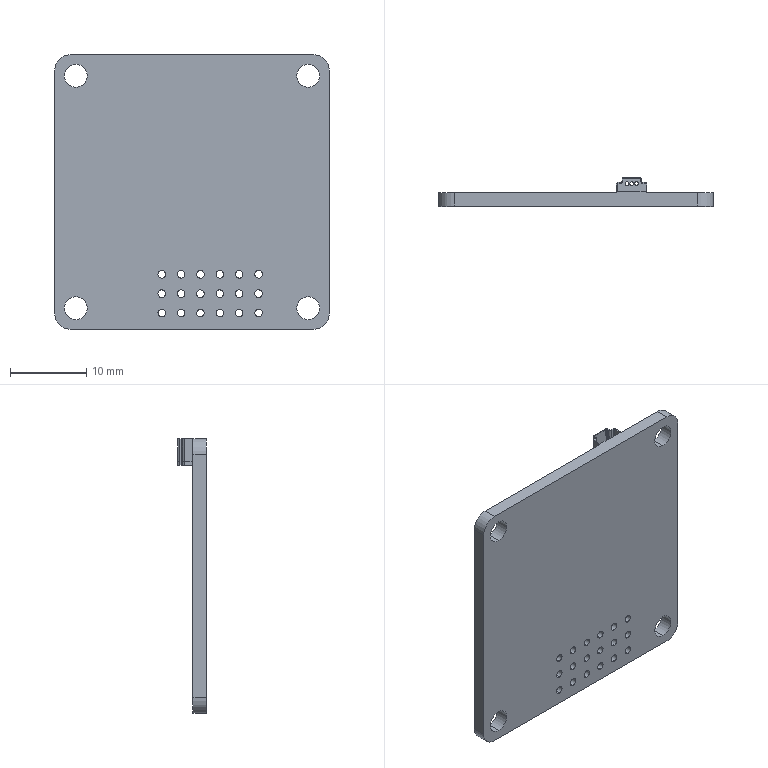Component | SolidWorks | 11.Distribution board-2 | 1 solid | 89 faces | box 36 x 3.75 x 36 mm | volume 2194 mm3 | cylinder 66 | plane 23 | commonest cylinder face diameters 1 x36 3 x8 0.486 x6 0.4 x6 4 x4 0.2 x4 0.6 x2
build123d program:
from build123d import *

# Parameters (mm, degrees)
SKETCH1_R               = 1.5
BOSS_EXTRUDE1_DEPTH     = 1.75
BOSS_EXTRUDE2_DEPTH     = 3
BOSS_EXTRUDE3_DEPTH     = 0.5
CUT_EXTRUDE1_REACH      = 39.34
SKETCH4_R               = 0.2432
CUT_EXTRUDE2_DEPTH      = 26.731
CUT_EXTRUDE2_DEPTH_BACK = 26.731
SKETCH5_R               = 0.5


with BuildPart() as part:
    # Sketch1 → Boss-Extrude1 (new body)
    with BuildSketch(Plane(origin=(0, 0, 0), x_dir=(1, 0, 0), z_dir=(0, 1, 0))):
        with BuildLine():
            Line((-16, -18), (16, -18))
            ThreePointArc((16, -18), (17.414, -17.414), (18, -16))
            Line((18, -16), (18, 16))
            ThreePointArc((18, 16), (17.414, 17.414), (16, 18))
            Line((16, 18), (-16, 18))
            ThreePointArc((-16, 18), (-17.414, 17.414), (-18, 16))
            Line((-18, 16), (-18, -16))
            ThreePointArc((-18, -16), (-17.414, -17.414), (-16, -18))
        make_face()
        with Locations(Location((-15.25, 15.25, 0), (0, 0, 270))):
            Circle(SKETCH1_R, mode=Mode.SUBTRACT)
        with Locations(Location((15.25, 15.25, 0), (0, 0, 270))):
            Circle(SKETCH1_R, mode=Mode.SUBTRACT)
        with Locations(Location((15.25, -15.25, 0), (0, 0, 270))):
            Circle(SKETCH1_R, mode=Mode.SUBTRACT)
        with Locations(Location((-15.25, -15.25, 0), (0, 0, 270))):
            Circle(SKETCH1_R, mode=Mode.SUBTRACT)
    extrude(amount=BOSS_EXTRUDE1_DEPTH)

    # Sketch2 → Boss-Extrude2 (add)
    with BuildSketch(Plane.XY.offset(18)):
        with BuildLine():
            Line((5.307, 1.75), (9.307, 1.75))
            Line((9.307, 1.75), (9.307, 2.894))
            ThreePointArc((9.307, 2.894), (9.248, 3.035), (9.107, 3.094))
            Line((9.107, 3.094), (8.767, 3.094))
            ThreePointArc((8.767, 3.094), (8.626, 3.152), (8.567, 3.294))
            Line((8.567, 3.294), (8.567, 3.55))
            ThreePointArc((8.567, 3.55), (8.508, 3.691), (8.367, 3.75))
            Line((8.367, 3.75), (6.247, 3.75))
            ThreePointArc((6.247, 3.75), (6.105, 3.691), (6.047, 3.55))
            Line((6.047, 3.55), (6.047, 3.294))
            ThreePointArc((6.047, 3.294), (5.988, 3.152), (5.847, 3.094))
            Line((5.847, 3.094), (5.507, 3.094))
            ThreePointArc((5.507, 3.094), (5.365, 3.035), (5.307, 2.894))
            Line((5.307, 2.894), (5.307, 1.75))
        make_face()
        with BuildLine():
            Line((6.247, 3.65), (8.367, 3.65))
            ThreePointArc((8.367, 3.65), (8.438, 3.621), (8.467, 3.55))
            Line((8.467, 3.55), (8.467, 3.294))
            ThreePointArc((8.467, 3.294), (8.555, 3.082), (8.767, 2.994))
            Line((8.767, 2.994), (9.107, 2.994))
            ThreePointArc((9.107, 2.994), (9.178, 2.965), (9.207, 2.894))
            Line((9.207, 2.894), (9.207, 1.85))
            Line((9.207, 1.85), (5.407, 1.85))
            Line((5.407, 1.85), (5.407, 2.894))
            ThreePointArc((5.407, 2.894), (5.436, 2.965), (5.507, 2.994))
            Line((5.507, 2.994), (5.847, 2.994))
            ThreePointArc((5.847, 2.994), (6.059, 3.082), (6.147, 3.294))
            Line((6.147, 3.294), (6.147, 3.55))
            ThreePointArc((6.147, 3.55), (6.176, 3.621), (6.247, 3.65))
        make_face(mode=Mode.SUBTRACT)
    extrude(amount=-BOSS_EXTRUDE2_DEPTH)

    # Sketch3 → Boss-Extrude3 (add)
    with BuildSketch(Plane(origin=(0, 0, 15), x_dir=(-1, 0, 0), z_dir=(0, 0, -1))):
        with BuildLine():
            Line((-5.307, 1.75), (-5.307, 2.894))
            ThreePointArc((-5.307, 2.894), (-5.365, 3.035), (-5.507, 3.094))
            Line((-5.507, 3.094), (-5.847, 3.094))
            ThreePointArc((-5.847, 3.094), (-5.988, 3.152), (-6.047, 3.294))
            Line((-6.047, 3.294), (-6.047, 3.55))
            ThreePointArc((-6.047, 3.55), (-6.105, 3.691), (-6.247, 3.75))
            Line((-6.247, 3.75), (-8.367, 3.75))
            ThreePointArc((-8.367, 3.75), (-8.508, 3.691), (-8.567, 3.55))
            Line((-8.567, 3.55), (-8.567, 3.294))
            ThreePointArc((-8.567, 3.294), (-8.626, 3.152), (-8.767, 3.094))
            Line((-8.767, 3.094), (-9.107, 3.094))
            ThreePointArc((-9.107, 3.094), (-9.248, 3.035), (-9.307, 2.894))
            Line((-9.307, 2.894), (-9.307, 1.75))
            Line((-9.307, 1.75), (-5.307, 1.75))
        make_face()
    extrude(amount=BOSS_EXTRUDE3_DEPTH)

    # Sketch4 → Cut-Extrude1 (cut, up to next)
    with BuildSketch(Plane(origin=(0, 0, 14.5), x_dir=(-1, 0, 0), z_dir=(0, 0, -1)), mode=Mode.PRIVATE) as cut_extrude1_sk1:
        with Locations((-7.307, 2.952)):
            Circle(SKETCH4_R)
    cut_extrude1_tool1 = extrude(cut_extrude1_sk1.sketch, amount=-CUT_EXTRUDE1_REACH, mode=Mode.PRIVATE) & part.part
    # Sketch4 → Cut-Extrude1 (cut, up to next)
    with BuildSketch(Plane(origin=(0, 0, 14.5), x_dir=(-1, 0, 0), z_dir=(0, 0, -1)), mode=Mode.PRIVATE) as cut_extrude1_sk2:
        with Locations((-6.69, 2.952)):
            Circle(SKETCH4_R)
    cut_extrude1_tool2 = extrude(cut_extrude1_sk2.sketch, amount=-CUT_EXTRUDE1_REACH, mode=Mode.PRIVATE) & part.part
    # Sketch4 → Cut-Extrude1 (cut, up to next)
    with BuildSketch(Plane(origin=(0, 0, 14.5), x_dir=(-1, 0, 0), z_dir=(0, 0, -1)), mode=Mode.PRIVATE) as cut_extrude1_sk3:
        with Locations((-7.932, 2.952)):
            Circle(SKETCH4_R)
    cut_extrude1_tool3 = extrude(cut_extrude1_sk3.sketch, amount=-CUT_EXTRUDE1_REACH, mode=Mode.PRIVATE) & part.part
    add(cut_extrude1_tool1.solids().sort_by_distance((7.307, 2.952, 14.5))[0], mode=Mode.SUBTRACT)
    add(cut_extrude1_tool2.solids().sort_by_distance((6.69, 2.952, 14.5))[0], mode=Mode.SUBTRACT)
    add(cut_extrude1_tool3.solids().sort_by_distance((7.932, 2.952, 14.5))[0], mode=Mode.SUBTRACT)

    # Sketch5 → Cut-Extrude2 (cut, two sides: drawn at the far end of the back side and taken through both)
    with BuildSketch(Plane.XZ.offset(-CUT_EXTRUDE2_DEPTH_BACK)):
        with Locations(Location((-3.97, -10.8, 0), (0, 0, 270))):
            Circle(SKETCH5_R)
        with Locations(Location((-3.97, -13.34, 0), (0, 0, 270))):
            Circle(SKETCH5_R)
        with Locations(Location((-3.97, -15.88, 0), (0, 0, 270))):
            Circle(SKETCH5_R)
        with Locations(Location((-1.43, -10.8, 0), (0, 0, 270))):
            Circle(SKETCH5_R)
        with Locations(Location((-1.43, -13.34, 0), (0, 0, 270))):
            Circle(SKETCH5_R)
        with Locations(Location((-1.43, -15.88, 0), (0, 0, 270))):
            Circle(SKETCH5_R)
        with Locations(Location((1.11, -10.8, 0), (0, 0, 270))):
            Circle(SKETCH5_R)
        with Locations(Location((1.11, -13.34, 0), (0, 0, 270))):
            Circle(SKETCH5_R)
        with Locations(Location((1.11, -15.88, 0), (0, 0, 270))):
            Circle(SKETCH5_R)
        with Locations(Location((3.65, -10.8, 0), (0, 0, 270))):
            Circle(SKETCH5_R)
        with Locations(Location((3.65, -13.34, 0), (0, 0, 270))):
            Circle(SKETCH5_R)
        with Locations(Location((3.65, -15.88, 0), (0, 0, 270))):
            Circle(SKETCH5_R)
        with Locations(Location((6.19, -10.8, 0), (0, 0, 270))):
            Circle(SKETCH5_R)
        with Locations(Location((6.19, -13.34, 0), (0, 0, 270))):
            Circle(SKETCH5_R)
        with Locations(Location((6.19, -15.88, 0), (0, 0, 270))):
            Circle(SKETCH5_R)
        with Locations(Location((8.73, -10.8, 0), (0, 0, 270))):
            Circle(SKETCH5_R)
        with Locations(Location((8.73, -13.34, 0), (0, 0, 270))):
            Circle(SKETCH5_R)
        with Locations(Location((8.73, -15.88, 0), (0, 0, 270))):
            Circle(SKETCH5_R)
    extrude(amount=CUT_EXTRUDE2_DEPTH + CUT_EXTRUDE2_DEPTH_BACK, mode=Mode.SUBTRACT)


solid = part.part

# Placed as in the assembly
solid = solid.moved(Location((0, 3.5, 0), (0, 0, 0)))